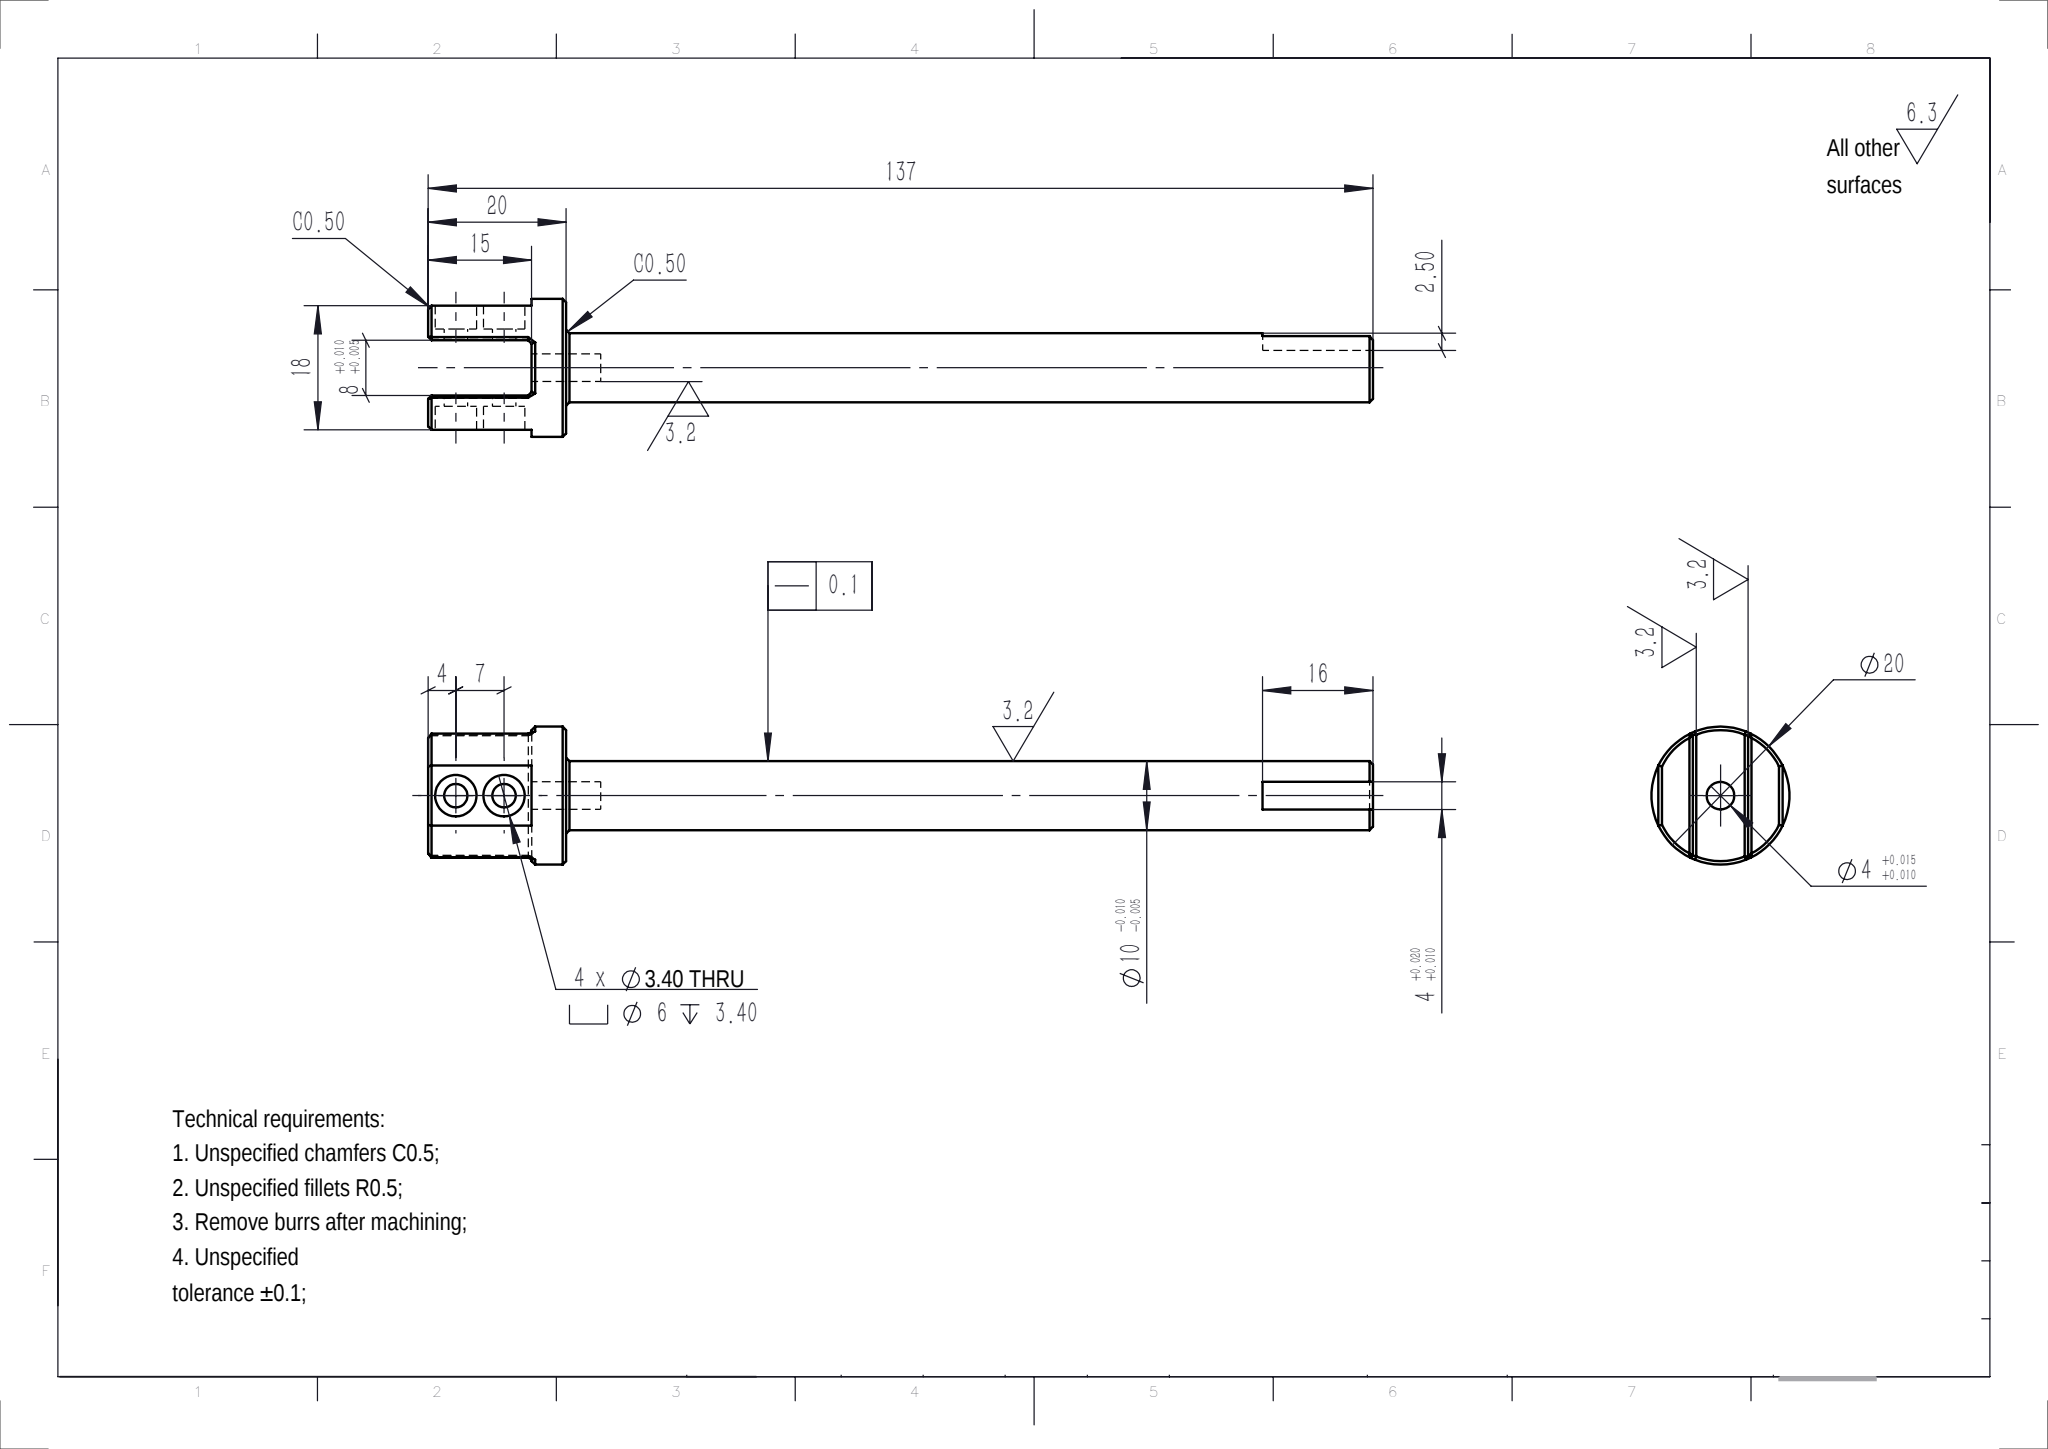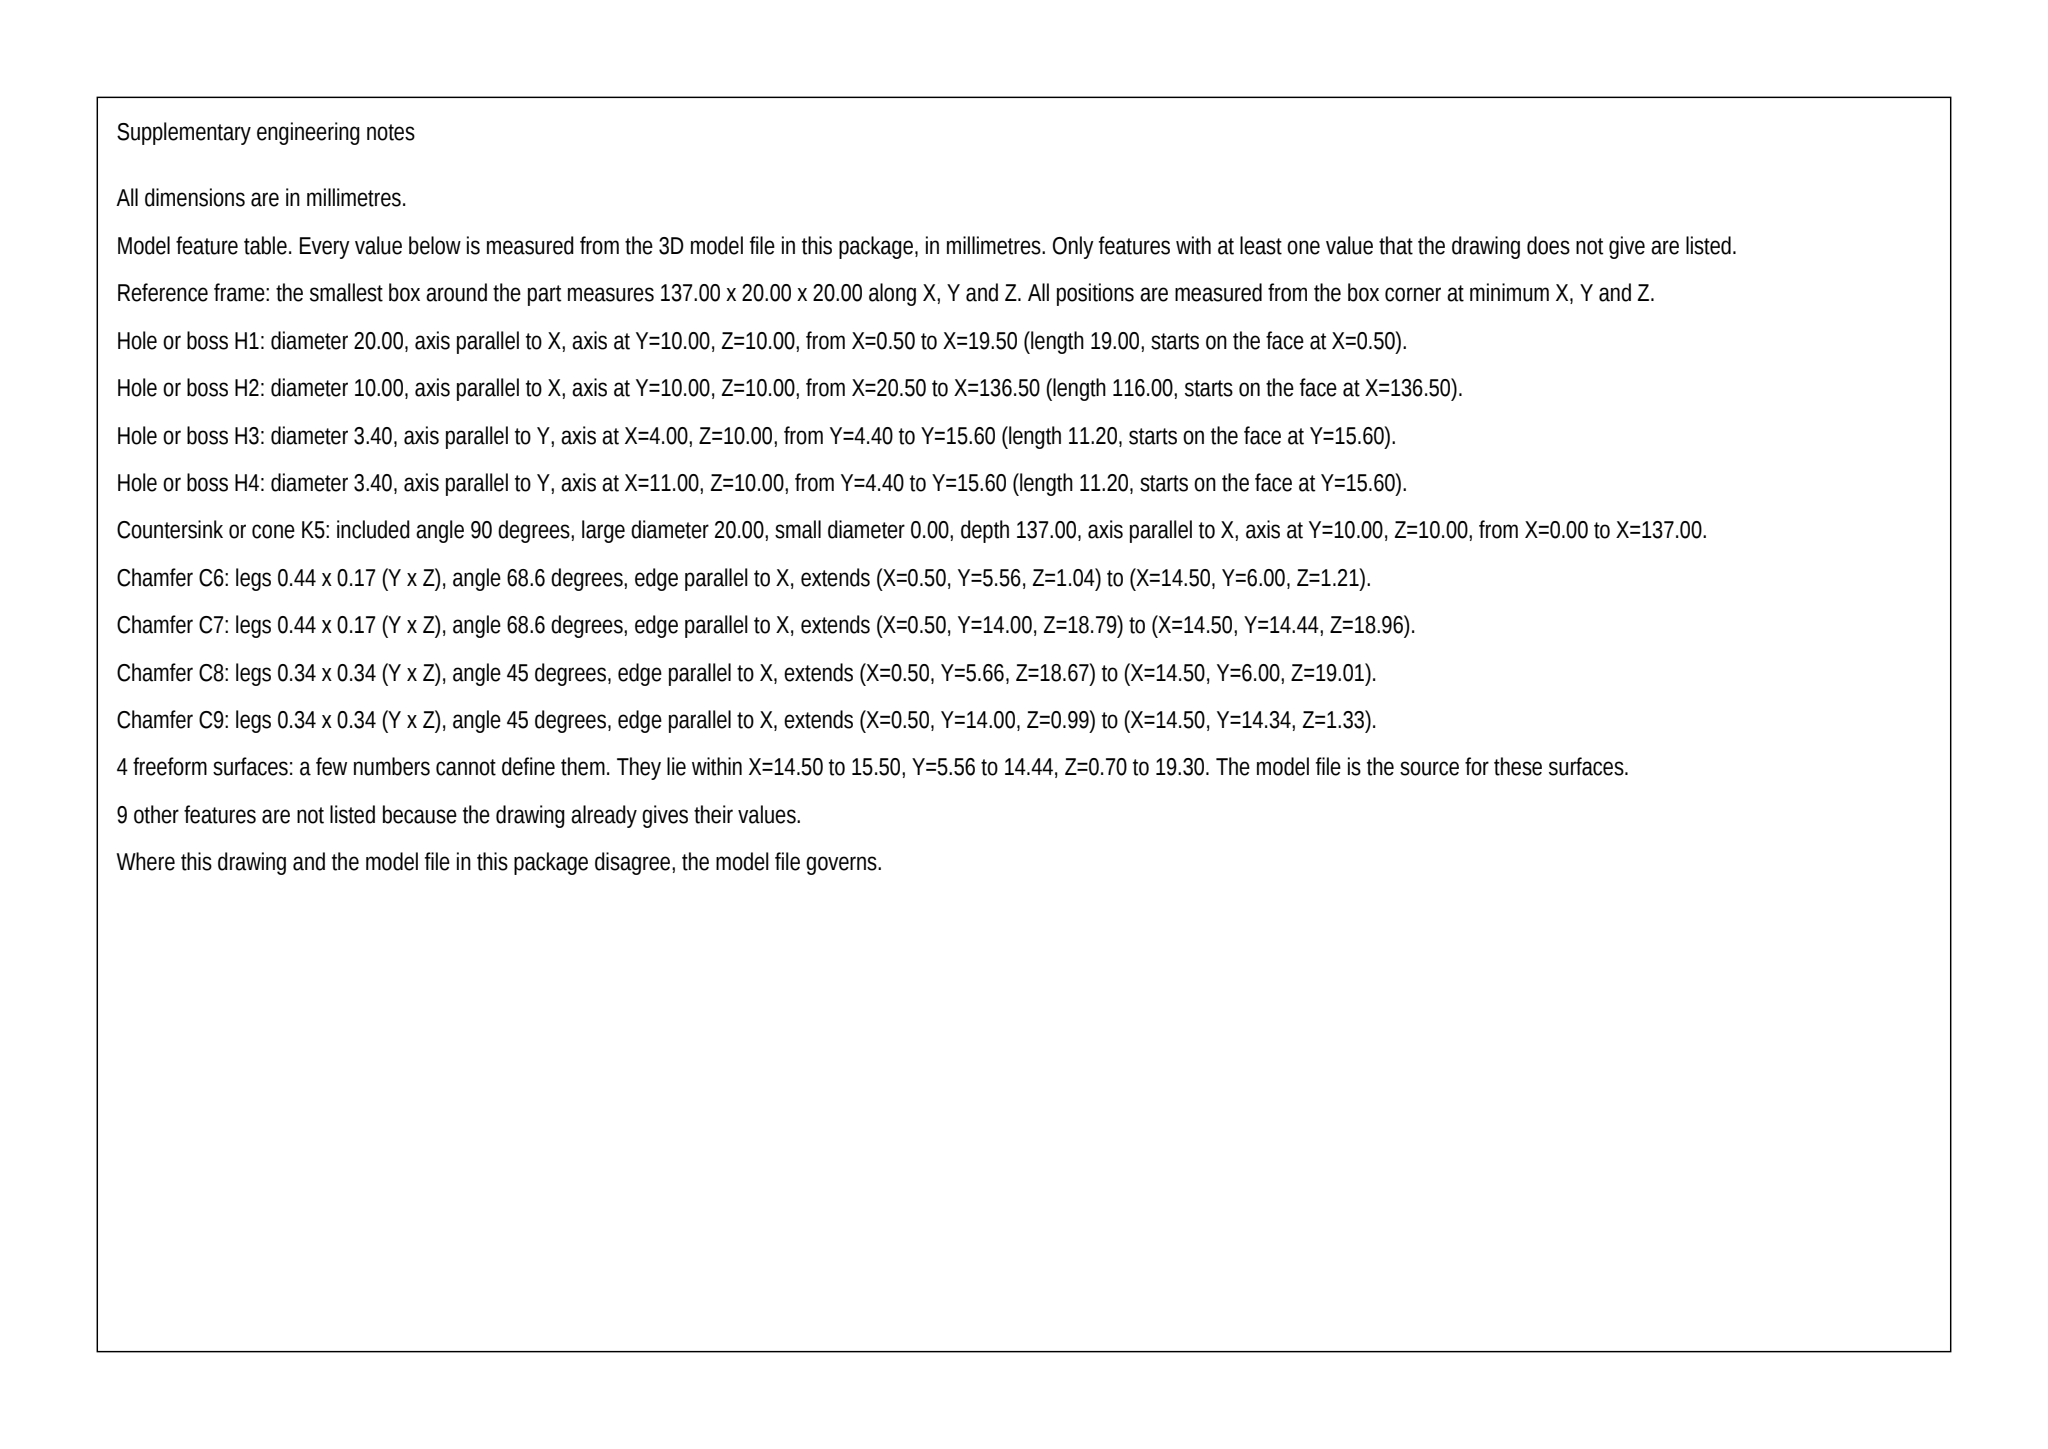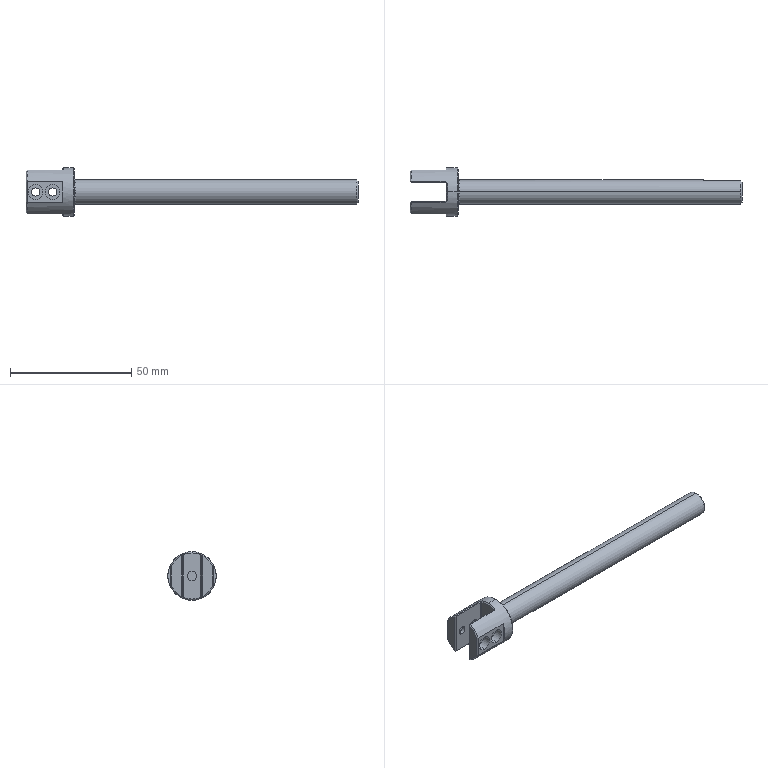Part | SolidWorks | mm | 1 solid | 74 faces | box 137 x 20 x 20 mm | volume 12223 mm3 | plane 34 | cylinder 22 | cone 14 | spline 4 | commonest cylinder face diameters 6 x8 3.4 x8 4 x2 10 x2 20 x2